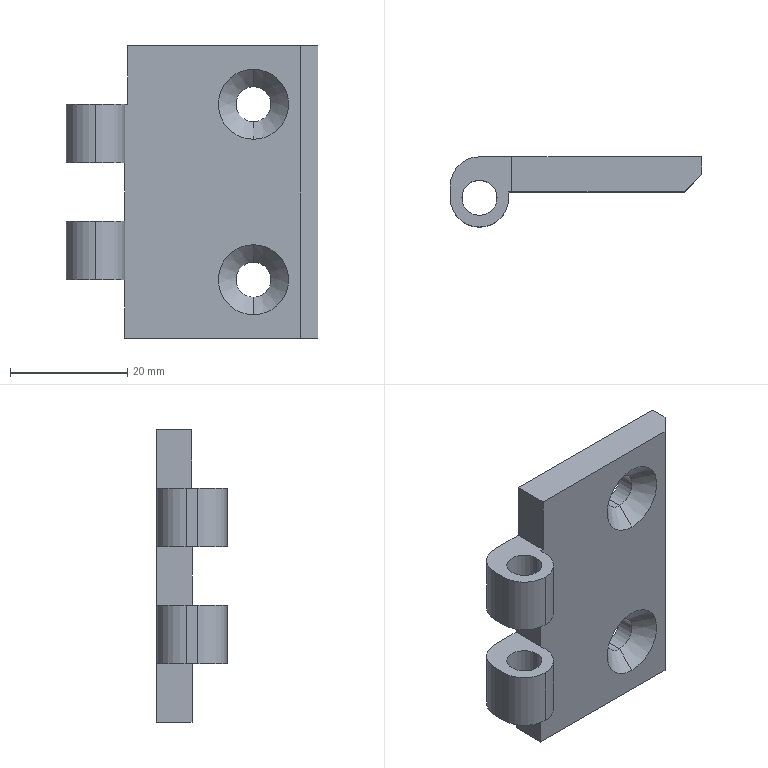Component | SolidWorks | OuterDoorHingeAssembly1-1_OuterHinge4-1 | 1 solid | 35 faces | box 43 x 12 x 50 mm | volume 10590 mm3 | plane 17 | cylinder 14 | cone 4 | commonest cylinder face diameters 6 x8 10 x6
STEP:
#1=COLOUR_RGB('',0.7922,0.8196,0.9333);
#2=FILL_AREA_STYLE_COLOUR('',#1);
#3=FILL_AREA_STYLE('',(#2));
#4=SURFACE_STYLE_FILL_AREA(#3);
#5=SURFACE_SIDE_STYLE('',(#4));
#6=SURFACE_STYLE_USAGE(.BOTH.,#5);
#7=PRESENTATION_STYLE_ASSIGNMENT((#6));
#8=CARTESIAN_POINT('',(3.383,-20.239,-59.646));
#9=VERTEX_POINT('',#8);
#10=CARTESIAN_POINT('',(3.383,-20.239,-59.409));
#11=VERTEX_POINT('',#10);
#12=CARTESIAN_POINT('',(3.383,-20.239,-59.528));
#13=DIRECTION('',(0.,-1.,0.));
#14=DIRECTION('',(-0.,0.,1.));
#15=AXIS2_PLACEMENT_3D('',#12,#13,#14);
#16=CIRCLE('',#15,0.1181);
#17=EDGE_CURVE('',#9,#11,#16,.T.);
#18=ORIENTED_EDGE('',*,*,#17,.F.);
#19=CARTESIAN_POINT('',(3.383,-20.357,-59.764));
#20=VERTEX_POINT('',#19);
#21=CARTESIAN_POINT('',(3.383,-20.239,-59.646));
#22=DIRECTION('',(0.,-0.7071,-0.7071));
#23=VECTOR('',#22,39.37);
#24=LINE('',#21,#23);
#25=EDGE_CURVE('',#9,#20,#24,.T.);
#26=ORIENTED_EDGE('',*,*,#25,.T.);
#27=CARTESIAN_POINT('',(3.383,-20.357,-59.291));
#28=VERTEX_POINT('',#27);
#29=CARTESIAN_POINT('',(3.383,-20.357,-59.528));
#30=DIRECTION('',(-0.,1.,-0.));
#31=DIRECTION('',(-0.,0.,1.));
#32=AXIS2_PLACEMENT_3D('',#29,#30,#31);
#33=CIRCLE('',#32,0.2362);
#34=EDGE_CURVE('',#28,#20,#33,.T.);
#35=ORIENTED_EDGE('',*,*,#34,.F.);
#36=CARTESIAN_POINT('',(3.383,-20.239,-59.409));
#37=DIRECTION('',(-0.,-0.7071,0.7071));
#38=VECTOR('',#37,39.37);
#39=LINE('',#36,#38);
#40=EDGE_CURVE('',#11,#28,#39,.T.);
#41=ORIENTED_EDGE('',*,*,#40,.F.);
#42=EDGE_LOOP('',(#18,#26,#35,#41));
#43=FACE_OUTER_BOUND('',#42,.T.);
#44=CARTESIAN_POINT('',(3.383,-20.239,-59.528));
#45=DIRECTION('',(0.,-1.,0.));
#46=DIRECTION('',(-0.,0.,1.));
#47=AXIS2_PLACEMENT_3D('',#44,#45,#46);
#48=CONICAL_SURFACE('',#47,0.1181,0.7854);
#49=ADVANCED_FACE('',(#43),#48,.F.);
#50=CARTESIAN_POINT('',(3.383,-20.239,-58.465));
#51=VERTEX_POINT('',#50);
#52=CARTESIAN_POINT('',(3.383,-20.239,-58.228));
#53=VERTEX_POINT('',#52);
#54=CARTESIAN_POINT('',(3.383,-20.239,-58.346));
#55=DIRECTION('',(0.,-1.,0.));
#56=DIRECTION('',(-0.,0.,1.));
#57=AXIS2_PLACEMENT_3D('',#54,#55,#56);
#58=CIRCLE('',#57,0.1181);
#59=EDGE_CURVE('',#51,#53,#58,.T.);
#60=ORIENTED_EDGE('',*,*,#59,.F.);
#61=CARTESIAN_POINT('',(3.383,-20.357,-58.583));
#62=VERTEX_POINT('',#61);
#63=CARTESIAN_POINT('',(3.383,-20.239,-58.465));
#64=DIRECTION('',(0.,-0.7071,-0.7071));
#65=VECTOR('',#64,39.37);
#66=LINE('',#63,#65);
#67=EDGE_CURVE('',#51,#62,#66,.T.);
#68=ORIENTED_EDGE('',*,*,#67,.T.);
#69=CARTESIAN_POINT('',(3.383,-20.357,-58.11));
#70=VERTEX_POINT('',#69);
#71=CARTESIAN_POINT('',(3.383,-20.357,-58.346));
#72=DIRECTION('',(-0.,1.,-0.));
#73=DIRECTION('',(-0.,0.,1.));
#74=AXIS2_PLACEMENT_3D('',#71,#72,#73);
#75=CIRCLE('',#74,0.2362);
#76=EDGE_CURVE('',#70,#62,#75,.T.);
#77=ORIENTED_EDGE('',*,*,#76,.F.);
#78=CARTESIAN_POINT('',(3.383,-20.239,-58.228));
#79=DIRECTION('',(-0.,-0.7071,0.7071));
#80=VECTOR('',#79,39.37);
#81=LINE('',#78,#80);
#82=EDGE_CURVE('',#53,#70,#81,.T.);
#83=ORIENTED_EDGE('',*,*,#82,.F.);
#84=EDGE_LOOP('',(#60,#68,#77,#83));
#85=FACE_OUTER_BOUND('',#84,.T.);
#86=CARTESIAN_POINT('',(3.383,-20.239,-58.346));
#87=DIRECTION('',(0.,-1.,0.));
#88=DIRECTION('',(-0.,0.,1.));
#89=AXIS2_PLACEMENT_3D('',#86,#87,#88);
#90=CONICAL_SURFACE('',#89,0.1181,0.7854);
#91=ADVANCED_FACE('',(#85),#90,.F.);
#92=CARTESIAN_POINT('',(3.383,-20.121,-59.646));
#93=VERTEX_POINT('',#92);
#94=CARTESIAN_POINT('',(3.383,-20.121,-59.409));
#95=VERTEX_POINT('',#94);
#96=CARTESIAN_POINT('',(3.383,-20.121,-59.528));
#97=DIRECTION('',(0.,-1.,0.));
#98=DIRECTION('',(-0.,0.,1.));
#99=AXIS2_PLACEMENT_3D('',#96,#97,#98);
#100=CIRCLE('',#99,0.1181);
#101=EDGE_CURVE('',#93,#95,#100,.T.);
#102=ORIENTED_EDGE('',*,*,#101,.F.);
#103=CARTESIAN_POINT('',(3.383,-19.964,-59.646));
#104=DIRECTION('',(0.,-1.,0.));
#105=VECTOR('',#104,39.37);
#106=LINE('',#103,#105);
#107=EDGE_CURVE('',#93,#9,#106,.T.);
#108=ORIENTED_EDGE('',*,*,#107,.T.);
#109=ORIENTED_EDGE('',*,*,#17,.T.);
#110=CARTESIAN_POINT('',(3.383,-19.964,-59.409));
#111=DIRECTION('',(0.,-1.,0.));
#112=VECTOR('',#111,39.37);
#113=LINE('',#110,#112);
#114=EDGE_CURVE('',#95,#11,#113,.T.);
#115=ORIENTED_EDGE('',*,*,#114,.F.);
#116=EDGE_LOOP('',(#102,#108,#109,#115));
#117=FACE_OUTER_BOUND('',#116,.T.);
#118=CARTESIAN_POINT('',(3.383,-19.964,-59.528));
#119=DIRECTION('',(0.,-1.,0.));
#120=DIRECTION('',(-0.,0.,1.));
#121=AXIS2_PLACEMENT_3D('',#118,#119,#120);
#122=CYLINDRICAL_SURFACE('',#121,0.1181);
#123=ADVANCED_FACE('',(#117),#122,.F.);
#124=CARTESIAN_POINT('',(3.383,-20.121,-58.465));
#125=VERTEX_POINT('',#124);
#126=CARTESIAN_POINT('',(3.383,-20.121,-58.228));
#127=VERTEX_POINT('',#126);
#128=CARTESIAN_POINT('',(3.383,-20.121,-58.346));
#129=DIRECTION('',(0.,-1.,0.));
#130=DIRECTION('',(-0.,0.,1.));
#131=AXIS2_PLACEMENT_3D('',#128,#129,#130);
#132=CIRCLE('',#131,0.1181);
#133=EDGE_CURVE('',#125,#127,#132,.T.);
#134=ORIENTED_EDGE('',*,*,#133,.F.);
#135=CARTESIAN_POINT('',(3.383,-19.964,-58.465));
#136=DIRECTION('',(0.,-1.,0.));
#137=VECTOR('',#136,39.37);
#138=LINE('',#135,#137);
#139=EDGE_CURVE('',#125,#51,#138,.T.);
#140=ORIENTED_EDGE('',*,*,#139,.T.);
#141=ORIENTED_EDGE('',*,*,#59,.T.);
#142=CARTESIAN_POINT('',(3.383,-19.964,-58.228));
#143=DIRECTION('',(0.,-1.,0.));
#144=VECTOR('',#143,39.37);
#145=LINE('',#142,#144);
#146=EDGE_CURVE('',#127,#53,#145,.T.);
#147=ORIENTED_EDGE('',*,*,#146,.F.);
#148=EDGE_LOOP('',(#134,#140,#141,#147));
#149=FACE_OUTER_BOUND('',#148,.T.);
#150=CARTESIAN_POINT('',(3.383,-19.964,-58.346));
#151=DIRECTION('',(0.,-1.,0.));
#152=DIRECTION('',(-0.,0.,1.));
#153=AXIS2_PLACEMENT_3D('',#150,#151,#152);
#154=CYLINDRICAL_SURFACE('',#153,0.1181);
#155=ADVANCED_FACE('',(#149),#154,.F.);
#156=CARTESIAN_POINT('',(2.202,-20.397,-59.528));
#157=VERTEX_POINT('',#156);
#158=CARTESIAN_POINT('',(2.438,-20.397,-59.528));
#159=VERTEX_POINT('',#158);
#160=CARTESIAN_POINT('',(2.32,-20.397,-59.528));
#161=DIRECTION('',(0.,-0.,-1.));
#162=DIRECTION('',(-1.,0.,0.));
#163=AXIS2_PLACEMENT_3D('',#160,#161,#162);
#164=CIRCLE('',#163,0.1181);
#165=EDGE_CURVE('',#157,#159,#164,.T.);
#166=ORIENTED_EDGE('',*,*,#165,.T.);
#167=CARTESIAN_POINT('',(2.438,-20.397,-59.134));
#168=VERTEX_POINT('',#167);
#169=CARTESIAN_POINT('',(2.438,-20.397,-60.315));
#170=DIRECTION('',(-0.,0.,1.));
#171=VECTOR('',#170,39.37);
#172=LINE('',#169,#171);
#173=EDGE_CURVE('',#159,#168,#172,.T.);
#174=ORIENTED_EDGE('',*,*,#173,.T.);
#175=CARTESIAN_POINT('',(2.202,-20.397,-59.134));
#176=VERTEX_POINT('',#175);
#177=CARTESIAN_POINT('',(2.32,-20.397,-59.134));
#178=DIRECTION('',(-0.,0.,1.));
#179=DIRECTION('',(1.,0.,0.));
#180=AXIS2_PLACEMENT_3D('',#177,#178,#179);
#181=CIRCLE('',#180,0.1181);
#182=EDGE_CURVE('',#168,#176,#181,.T.);
#183=ORIENTED_EDGE('',*,*,#182,.T.);
#184=CARTESIAN_POINT('',(2.202,-20.397,-60.315));
#185=DIRECTION('',(-0.,0.,1.));
#186=VECTOR('',#185,39.37);
#187=LINE('',#184,#186);
#188=EDGE_CURVE('',#157,#176,#187,.T.);
#189=ORIENTED_EDGE('',*,*,#188,.F.);
#190=EDGE_LOOP('',(#166,#174,#183,#189));
#191=FACE_OUTER_BOUND('',#190,.T.);
#192=CARTESIAN_POINT('',(2.32,-20.397,-60.315));
#193=DIRECTION('',(-0.,0.,1.));
#194=DIRECTION('',(-1.,0.,0.));
#195=AXIS2_PLACEMENT_3D('',#192,#193,#194);
#196=CYLINDRICAL_SURFACE('',#195,0.1181);
#197=ADVANCED_FACE('',(#191),#196,.F.);
#198=CARTESIAN_POINT('',(2.202,-20.397,-58.74));
#199=VERTEX_POINT('',#198);
#200=CARTESIAN_POINT('',(2.438,-20.397,-58.74));
#201=VERTEX_POINT('',#200);
#202=CARTESIAN_POINT('',(2.32,-20.397,-58.74));
#203=DIRECTION('',(0.,-0.,-1.));
#204=DIRECTION('',(-1.,0.,0.));
#205=AXIS2_PLACEMENT_3D('',#202,#203,#204);
#206=CIRCLE('',#205,0.1181);
#207=EDGE_CURVE('',#199,#201,#206,.T.);
#208=ORIENTED_EDGE('',*,*,#207,.T.);
#209=CARTESIAN_POINT('',(2.438,-20.397,-58.346));
#210=VERTEX_POINT('',#209);
#211=CARTESIAN_POINT('',(2.438,-20.397,-60.315));
#212=DIRECTION('',(-0.,0.,1.));
#213=VECTOR('',#212,39.37);
#214=LINE('',#211,#213);
#215=EDGE_CURVE('',#201,#210,#214,.T.);
#216=ORIENTED_EDGE('',*,*,#215,.T.);
#217=CARTESIAN_POINT('',(2.202,-20.397,-58.346));
#218=VERTEX_POINT('',#217);
#219=CARTESIAN_POINT('',(2.32,-20.397,-58.346));
#220=DIRECTION('',(-0.,0.,1.));
#221=DIRECTION('',(1.,0.,0.));
#222=AXIS2_PLACEMENT_3D('',#219,#220,#221);
#223=CIRCLE('',#222,0.1181);
#224=EDGE_CURVE('',#210,#218,#223,.T.);
#225=ORIENTED_EDGE('',*,*,#224,.T.);
#226=CARTESIAN_POINT('',(2.202,-20.397,-60.315));
#227=DIRECTION('',(-0.,0.,1.));
#228=VECTOR('',#227,39.37);
#229=LINE('',#226,#228);
#230=EDGE_CURVE('',#199,#218,#229,.T.);
#231=ORIENTED_EDGE('',*,*,#230,.F.);
#232=EDGE_LOOP('',(#208,#216,#225,#231));
#233=FACE_OUTER_BOUND('',#232,.T.);
#234=CARTESIAN_POINT('',(2.32,-20.397,-60.315));
#235=DIRECTION('',(-0.,0.,1.));
#236=DIRECTION('',(-1.,0.,0.));
#237=AXIS2_PLACEMENT_3D('',#234,#235,#236);
#238=CYLINDRICAL_SURFACE('',#237,0.1181);
#239=ADVANCED_FACE('',(#233),#238,.F.);
#240=CARTESIAN_POINT('',(2.123,-20.397,-58.74));
#241=VERTEX_POINT('',#240);
#242=CARTESIAN_POINT('',(2.123,-20.397,-58.346));
#243=VERTEX_POINT('',#242);
#244=CARTESIAN_POINT('',(2.123,-20.397,-59.921));
#245=DIRECTION('',(-0.,0.,1.));
#246=VECTOR('',#245,39.37);
#247=LINE('',#244,#246);
#248=EDGE_CURVE('',#241,#243,#247,.T.);
#249=ORIENTED_EDGE('',*,*,#248,.T.);
#250=CARTESIAN_POINT('',(2.123,-20.318,-58.346));
#251=VERTEX_POINT('',#250);
#252=CARTESIAN_POINT('',(2.123,-20.357,-58.346));
#253=DIRECTION('',(-0.,1.,-0.));
#254=VECTOR('',#253,39.37);
#255=LINE('',#252,#254);
#256=EDGE_CURVE('',#243,#251,#255,.T.);
#257=ORIENTED_EDGE('',*,*,#256,.T.);
#258=CARTESIAN_POINT('',(2.123,-20.318,-58.74));
#259=VERTEX_POINT('',#258);
#260=CARTESIAN_POINT('',(2.123,-20.318,-59.921));
#261=DIRECTION('',(0.,-0.,-1.));
#262=VECTOR('',#261,39.37);
#263=LINE('',#260,#262);
#264=EDGE_CURVE('',#251,#259,#263,.T.);
#265=ORIENTED_EDGE('',*,*,#264,.T.);
#266=CARTESIAN_POINT('',(2.123,-20.357,-58.74));
#267=DIRECTION('',(0.,-1.,0.));
#268=VECTOR('',#267,39.37);
#269=LINE('',#266,#268);
#270=EDGE_CURVE('',#259,#241,#269,.T.);
#271=ORIENTED_EDGE('',*,*,#270,.T.);
#272=EDGE_LOOP('',(#249,#257,#265,#271));
#273=FACE_OUTER_BOUND('',#272,.T.);
#274=CARTESIAN_POINT('',(2.123,-20.357,-59.921));
#275=DIRECTION('',(1.,0.,0.));
#276=DIRECTION('',(-0.,0.,1.));
#277=AXIS2_PLACEMENT_3D('',#274,#275,#276);
#278=PLANE('',#277);
#279=ADVANCED_FACE('',(#273),#278,.F.);
#280=CARTESIAN_POINT('',(2.517,-20.357,-58.74));
#281=VERTEX_POINT('',#280);
#282=CARTESIAN_POINT('',(2.517,-20.357,-58.346));
#283=VERTEX_POINT('',#282);
#284=CARTESIAN_POINT('',(2.517,-20.357,-59.921));
#285=DIRECTION('',(-0.,0.,1.));
#286=VECTOR('',#285,39.37);
#287=LINE('',#284,#286);
#288=EDGE_CURVE('',#281,#283,#287,.T.);
#289=ORIENTED_EDGE('',*,*,#288,.T.);
#290=CARTESIAN_POINT('',(2.517,-20.397,-58.346));
#291=VERTEX_POINT('',#290);
#292=CARTESIAN_POINT('',(2.517,-20.594,-58.346));
#293=DIRECTION('',(0.,-1.,0.));
#294=VECTOR('',#293,39.37);
#295=LINE('',#292,#294);
#296=EDGE_CURVE('',#283,#291,#295,.T.);
#297=ORIENTED_EDGE('',*,*,#296,.T.);
#298=CARTESIAN_POINT('',(2.517,-20.397,-58.74));
#299=VERTEX_POINT('',#298);
#300=CARTESIAN_POINT('',(2.517,-20.397,-59.921));
#301=DIRECTION('',(0.,-0.,-1.));
#302=VECTOR('',#301,39.37);
#303=LINE('',#300,#302);
#304=EDGE_CURVE('',#291,#299,#303,.T.);
#305=ORIENTED_EDGE('',*,*,#304,.T.);
#306=CARTESIAN_POINT('',(2.517,-20.712,-58.74));
#307=DIRECTION('',(-0.,1.,-0.));
#308=VECTOR('',#307,39.37);
#309=LINE('',#306,#308);
#310=EDGE_CURVE('',#299,#281,#309,.T.);
#311=ORIENTED_EDGE('',*,*,#310,.T.);
#312=EDGE_LOOP('',(#289,#297,#305,#311));
#313=FACE_OUTER_BOUND('',#312,.T.);
#314=CARTESIAN_POINT('',(2.517,-20.594,-59.921));
#315=DIRECTION('',(-1.,-0.,-0.));
#316=DIRECTION('',(0.,-0.,-1.));
#317=AXIS2_PLACEMENT_3D('',#314,#315,#316);
#318=PLANE('',#317);
#319=ADVANCED_FACE('',(#313),#318,.F.);
#320=ORIENTED_EDGE('',*,*,#215,.F.);
#321=CARTESIAN_POINT('',(2.32,-20.397,-58.74));
#322=DIRECTION('',(0.,-0.,-1.));
#323=DIRECTION('',(-1.,0.,0.));
#324=AXIS2_PLACEMENT_3D('',#321,#322,#323);
#325=CIRCLE('',#324,0.1181);
#326=EDGE_CURVE('',#201,#199,#325,.T.);
#327=ORIENTED_EDGE('',*,*,#326,.T.);
#328=ORIENTED_EDGE('',*,*,#230,.T.);
#329=CARTESIAN_POINT('',(2.32,-20.397,-58.346));
#330=DIRECTION('',(-0.,0.,1.));
#331=DIRECTION('',(1.,0.,0.));
#332=AXIS2_PLACEMENT_3D('',#329,#330,#331);
#333=CIRCLE('',#332,0.1181);
#334=EDGE_CURVE('',#218,#210,#333,.T.);
#335=ORIENTED_EDGE('',*,*,#334,.T.);
#336=EDGE_LOOP('',(#320,#327,#328,#335));
#337=FACE_OUTER_BOUND('',#336,.T.);
#338=CARTESIAN_POINT('',(2.32,-20.397,-60.315));
#339=DIRECTION('',(-0.,0.,1.));
#340=DIRECTION('',(-1.,0.,0.));
#341=AXIS2_PLACEMENT_3D('',#338,#339,#340);
#342=CYLINDRICAL_SURFACE('',#341,0.1181);
#343=ADVANCED_FACE('',(#337),#342,.F.);
#344=CARTESIAN_POINT('',(2.32,-20.121,-58.346));
#345=VERTEX_POINT('',#344);
#346=CARTESIAN_POINT('',(2.32,-20.318,-58.346));
#347=DIRECTION('',(-0.,0.,1.));
#348=DIRECTION('',(1.,0.,0.));
#349=AXIS2_PLACEMENT_3D('',#346,#347,#348);
#350=CIRCLE('',#349,0.1969);
#351=EDGE_CURVE('',#345,#251,#350,.T.);
#352=ORIENTED_EDGE('',*,*,#351,.F.);
#353=CARTESIAN_POINT('',(2.32,-20.121,-58.74));
#354=VERTEX_POINT('',#353);
#355=CARTESIAN_POINT('',(2.32,-20.121,-57.953));
#356=DIRECTION('',(-0.,0.,1.));
#357=VECTOR('',#356,39.37);
#358=LINE('',#355,#357);
#359=EDGE_CURVE('',#354,#345,#358,.T.);
#360=ORIENTED_EDGE('',*,*,#359,.F.);
#361=CARTESIAN_POINT('',(2.32,-20.318,-58.74));
#362=DIRECTION('',(0.,-0.,-1.));
#363=DIRECTION('',(-1.,0.,0.));
#364=AXIS2_PLACEMENT_3D('',#361,#362,#363);
#365=CIRCLE('',#364,0.1969);
#366=EDGE_CURVE('',#259,#354,#365,.T.);
#367=ORIENTED_EDGE('',*,*,#366,.F.);
#368=ORIENTED_EDGE('',*,*,#264,.F.);
#369=EDGE_LOOP('',(#352,#360,#367,#368));
#370=FACE_OUTER_BOUND('',#369,.T.);
#371=CARTESIAN_POINT('',(2.32,-20.318,-59.921));
#372=DIRECTION('',(0.,-0.,-1.));
#373=DIRECTION('',(1.,0.,0.));
#374=AXIS2_PLACEMENT_3D('',#371,#372,#373);
#375=CYLINDRICAL_SURFACE('',#374,0.1969);
#376=ADVANCED_FACE('',(#370),#375,.T.);
#377=CARTESIAN_POINT('',(2.32,-20.594,-58.346));
#378=VERTEX_POINT('',#377);
#379=CARTESIAN_POINT('',(2.32,-20.397,-58.346));
#380=DIRECTION('',(-0.,0.,1.));
#381=DIRECTION('',(1.,0.,0.));
#382=AXIS2_PLACEMENT_3D('',#379,#380,#381);
#383=CIRCLE('',#382,0.1969);
#384=EDGE_CURVE('',#243,#378,#383,.T.);
#385=ORIENTED_EDGE('',*,*,#384,.F.);
#386=ORIENTED_EDGE('',*,*,#248,.F.);
#387=CARTESIAN_POINT('',(2.32,-20.594,-58.74));
#388=VERTEX_POINT('',#387);
#389=CARTESIAN_POINT('',(2.32,-20.397,-58.74));
#390=DIRECTION('',(0.,-0.,-1.));
#391=DIRECTION('',(-1.,0.,0.));
#392=AXIS2_PLACEMENT_3D('',#389,#390,#391);
#393=CIRCLE('',#392,0.1969);
#394=EDGE_CURVE('',#388,#241,#393,.T.);
#395=ORIENTED_EDGE('',*,*,#394,.F.);
#396=CARTESIAN_POINT('',(2.32,-20.594,-57.953));
#397=DIRECTION('',(0.,-0.,-1.));
#398=VECTOR('',#397,39.37);
#399=LINE('',#396,#398);
#400=EDGE_CURVE('',#378,#388,#399,.T.);
#401=ORIENTED_EDGE('',*,*,#400,.F.);
#402=EDGE_LOOP('',(#385,#386,#395,#401));
#403=FACE_OUTER_BOUND('',#402,.T.);
#404=CARTESIAN_POINT('',(2.32,-20.397,-57.953));
#405=DIRECTION('',(0.,-0.,-1.));
#406=DIRECTION('',(1.,0.,0.));
#407=AXIS2_PLACEMENT_3D('',#404,#405,#406);
#408=CYLINDRICAL_SURFACE('',#407,0.1969);
#409=ADVANCED_FACE('',(#403),#408,.T.);
#410=CARTESIAN_POINT('',(2.32,-20.397,-58.346));
#411=DIRECTION('',(-0.,0.,1.));
#412=DIRECTION('',(1.,0.,0.));
#413=AXIS2_PLACEMENT_3D('',#410,#411,#412);
#414=CIRCLE('',#413,0.1969);
#415=EDGE_CURVE('',#378,#291,#414,.T.);
#416=ORIENTED_EDGE('',*,*,#415,.F.);
#417=ORIENTED_EDGE('',*,*,#400,.T.);
#418=CARTESIAN_POINT('',(2.32,-20.397,-58.74));
#419=DIRECTION('',(0.,-0.,-1.));
#420=DIRECTION('',(-1.,0.,0.));
#421=AXIS2_PLACEMENT_3D('',#418,#419,#420);
#422=CIRCLE('',#421,0.1969);
#423=EDGE_CURVE('',#299,#388,#422,.T.);
#424=ORIENTED_EDGE('',*,*,#423,.F.);
#425=ORIENTED_EDGE('',*,*,#304,.F.);
#426=EDGE_LOOP('',(#416,#417,#424,#425));
#427=FACE_OUTER_BOUND('',#426,.T.);
#428=CARTESIAN_POINT('',(2.32,-20.397,-57.953));
#429=DIRECTION('',(-0.,0.,1.));
#430=DIRECTION('',(-1.,0.,0.));
#431=AXIS2_PLACEMENT_3D('',#428,#429,#430);
#432=CYLINDRICAL_SURFACE('',#431,0.1969);
#433=ADVANCED_FACE('',(#427),#432,.T.);
#434=CARTESIAN_POINT('',(3.816,-20.239,-57.953));
#435=VERTEX_POINT('',#434);
#436=CARTESIAN_POINT('',(3.816,-20.121,-57.953));
#437=VERTEX_POINT('',#436);
#438=CARTESIAN_POINT('',(3.816,-20.357,-57.953));
#439=DIRECTION('',(-0.,1.,-0.));
#440=VECTOR('',#439,39.37);
#441=LINE('',#438,#440);
#442=EDGE_CURVE('',#435,#437,#441,.T.);
#443=ORIENTED_EDGE('',*,*,#442,.F.);
#444=CARTESIAN_POINT('',(3.816,-20.239,-59.921));
#445=VERTEX_POINT('',#444);
#446=CARTESIAN_POINT('',(3.816,-20.239,-59.921));
#447=DIRECTION('',(0.,-0.,-1.));
#448=VECTOR('',#447,39.37);
#449=LINE('',#446,#448);
#450=EDGE_CURVE('',#435,#445,#449,.T.);
#451=ORIENTED_EDGE('',*,*,#450,.T.);
#452=CARTESIAN_POINT('',(3.816,-20.121,-59.921));
#453=VERTEX_POINT('',#452);
#454=CARTESIAN_POINT('',(3.816,-20.357,-59.921));
#455=DIRECTION('',(-0.,1.,-0.));
#456=VECTOR('',#455,39.37);
#457=LINE('',#454,#456);
#458=EDGE_CURVE('',#445,#453,#457,.T.);
#459=ORIENTED_EDGE('',*,*,#458,.T.);
#460=CARTESIAN_POINT('',(3.816,-20.121,-59.921));
#461=DIRECTION('',(-0.,0.,1.));
#462=VECTOR('',#461,39.37);
#463=LINE('',#460,#462);
#464=EDGE_CURVE('',#453,#437,#463,.T.);
#465=ORIENTED_EDGE('',*,*,#464,.T.);
#466=EDGE_LOOP('',(#443,#451,#459,#465));
#467=FACE_OUTER_BOUND('',#466,.T.);
#468=CARTESIAN_POINT('',(3.816,-20.357,-59.921));
#469=DIRECTION('',(-1.,-0.,-0.));
#470=DIRECTION('',(0.,-0.,-1.));
#471=AXIS2_PLACEMENT_3D('',#468,#469,#470);
#472=PLANE('',#471);
#473=ADVANCED_FACE('',(#467),#472,.F.);
#474=CARTESIAN_POINT('',(3.698,-20.357,-57.953));
#475=VERTEX_POINT('',#474);
#476=CARTESIAN_POINT('',(2.538,-20.357,-57.953));
#477=VERTEX_POINT('',#476);
#478=CARTESIAN_POINT('',(3.816,-20.357,-57.953));
#479=DIRECTION('',(-1.,-0.,-0.));
#480=VECTOR('',#479,39.37);
#481=LINE('',#478,#480);
#482=EDGE_CURVE('',#475,#477,#481,.T.);
#483=ORIENTED_EDGE('',*,*,#482,.F.);
#484=CARTESIAN_POINT('',(3.698,-20.357,-57.953));
#485=DIRECTION('',(0.7071,0.7071,0.));
#486=VECTOR('',#485,39.37);
#487=LINE('',#484,#486);
#488=EDGE_CURVE('',#475,#435,#487,.T.);
#489=ORIENTED_EDGE('',*,*,#488,.T.);
#490=ORIENTED_EDGE('',*,*,#442,.T.);
#491=CARTESIAN_POINT('',(2.538,-20.121,-57.953));
#492=VERTEX_POINT('',#491);
#493=CARTESIAN_POINT('',(3.816,-20.121,-57.953));
#494=DIRECTION('',(-1.,-0.,-0.));
#495=VECTOR('',#494,39.37);
#496=LINE('',#493,#495);
#497=EDGE_CURVE('',#437,#492,#496,.T.);
#498=ORIENTED_EDGE('',*,*,#497,.T.);
#499=CARTESIAN_POINT('',(2.538,-20.357,-57.953));
#500=DIRECTION('',(0.,-1.,0.));
#501=VECTOR('',#500,39.37);
#502=LINE('',#499,#501);
#503=EDGE_CURVE('',#492,#477,#502,.T.);
#504=ORIENTED_EDGE('',*,*,#503,.T.);
#505=EDGE_LOOP('',(#483,#489,#490,#498,#504));
#506=FACE_OUTER_BOUND('',#505,.T.);
#507=CARTESIAN_POINT('',(3.816,-20.357,-57.953));
#508=DIRECTION('',(0.,-0.,-1.));
#509=DIRECTION('',(1.,0.,0.));
#510=AXIS2_PLACEMENT_3D('',#507,#508,#509);
#511=PLANE('',#510);
#512=ADVANCED_FACE('',(#506),#511,.F.);
#513=CARTESIAN_POINT('',(2.123,-20.397,-59.528));
#514=VERTEX_POINT('',#513);
#515=CARTESIAN_POINT('',(2.123,-20.397,-59.134));
#516=VERTEX_POINT('',#515);
#517=CARTESIAN_POINT('',(2.123,-20.397,-59.921));
#518=DIRECTION('',(-0.,0.,1.));
#519=VECTOR('',#518,39.37);
#520=LINE('',#517,#519);
#521=EDGE_CURVE('',#514,#516,#520,.T.);
#522=ORIENTED_EDGE('',*,*,#521,.T.);
#523=CARTESIAN_POINT('',(2.123,-20.318,-59.134));
#524=VERTEX_POINT('',#523);
#525=CARTESIAN_POINT('',(2.123,-20.357,-59.134));
#526=DIRECTION('',(-0.,1.,-0.));
#527=VECTOR('',#526,39.37);
#528=LINE('',#525,#527);
#529=EDGE_CURVE('',#516,#524,#528,.T.);
#530=ORIENTED_EDGE('',*,*,#529,.T.);
#531=CARTESIAN_POINT('',(2.123,-20.318,-59.528));
#532=VERTEX_POINT('',#531);
#533=CARTESIAN_POINT('',(2.123,-20.318,-59.921));
#534=DIRECTION('',(0.,-0.,-1.));
#535=VECTOR('',#534,39.37);
#536=LINE('',#533,#535);
#537=EDGE_CURVE('',#524,#532,#536,.T.);
#538=ORIENTED_EDGE('',*,*,#537,.T.);
#539=CARTESIAN_POINT('',(2.123,-20.357,-59.528));
#540=DIRECTION('',(0.,-1.,0.));
#541=VECTOR('',#540,39.37);
#542=LINE('',#539,#541);
#543=EDGE_CURVE('',#532,#514,#542,.T.);
#544=ORIENTED_EDGE('',*,*,#543,.T.);
#545=EDGE_LOOP('',(#522,#530,#538,#544));
#546=FACE_OUTER_BOUND('',#545,.T.);
#547=CARTESIAN_POINT('',(2.123,-20.357,-59.921));
#548=DIRECTION('',(1.,0.,0.));
#549=DIRECTION('',(-0.,0.,1.));
#550=AXIS2_PLACEMENT_3D('',#547,#548,#549);
#551=PLANE('',#550);
#552=ADVANCED_FACE('',(#546),#551,.F.);
#553=ORIENTED_EDGE('',*,*,#458,.F.);
#554=CARTESIAN_POINT('',(3.698,-20.357,-59.921));
#555=VERTEX_POINT('',#554);
#556=CARTESIAN_POINT('',(3.698,-20.357,-59.921));
#557=DIRECTION('',(-0.7071,-0.7071,-0.));
#558=VECTOR('',#557,39.37);
#559=LINE('',#556,#558);
#560=EDGE_CURVE('',#445,#555,#559,.T.);
#561=ORIENTED_EDGE('',*,*,#560,.T.);
#562=CARTESIAN_POINT('',(2.517,-20.357,-59.921));
#563=VERTEX_POINT('',#562);
#564=CARTESIAN_POINT('',(3.816,-20.357,-59.921));
#565=DIRECTION('',(1.,0.,0.));
#566=VECTOR('',#565,39.37);
#567=LINE('',#564,#566);
#568=EDGE_CURVE('',#563,#555,#567,.T.);
#569=ORIENTED_EDGE('',*,*,#568,.F.);
#570=CARTESIAN_POINT('',(2.517,-20.121,-59.921));
#571=VERTEX_POINT('',#570);
#572=CARTESIAN_POINT('',(2.517,-20.712,-59.921));
#573=DIRECTION('',(-0.,1.,-0.));
#574=VECTOR('',#573,39.37);
#575=LINE('',#572,#574);
#576=EDGE_CURVE('',#563,#571,#575,.T.);
#577=ORIENTED_EDGE('',*,*,#576,.T.);
#578=CARTESIAN_POINT('',(3.816,-20.121,-59.921));
#579=DIRECTION('',(1.,0.,0.));
#580=VECTOR('',#579,39.37);
#581=LINE('',#578,#580);
#582=EDGE_CURVE('',#571,#453,#581,.T.);
#583=ORIENTED_EDGE('',*,*,#582,.T.);
#584=EDGE_LOOP('',(#553,#561,#569,#577,#583));
#585=FACE_OUTER_BOUND('',#584,.T.);
#586=CARTESIAN_POINT('',(3.816,-20.357,-59.921));
#587=DIRECTION('',(-0.,0.,1.));
#588=DIRECTION('',(-1.,-0.,-0.));
#589=AXIS2_PLACEMENT_3D('',#586,#587,#588);
#590=PLANE('',#589);
#591=ADVANCED_FACE('',(#585),#590,.F.);
#592=ORIENTED_EDGE('',*,*,#76,.T.);
#593=CARTESIAN_POINT('',(3.383,-20.357,-58.346));
#594=DIRECTION('',(-0.,1.,-0.));
#595=DIRECTION('',(-0.,0.,1.));
#596=AXIS2_PLACEMENT_3D('',#593,#594,#595);
#597=CIRCLE('',#596,0.2362);
#598=EDGE_CURVE('',#62,#70,#597,.T.);
#599=ORIENTED_EDGE('',*,*,#598,.T.);
#600=EDGE_LOOP('',(#592,#599));
#601=FACE_BOUND('',#600,.T.);
#602=ORIENTED_EDGE('',*,*,#34,.T.);
#603=CARTESIAN_POINT('',(3.383,-20.357,-59.528));
#604=DIRECTION('',(-0.,1.,-0.));
#605=DIRECTION('',(-0.,0.,1.));
#606=AXIS2_PLACEMENT_3D('',#603,#604,#605);
#607=CIRCLE('',#606,0.2362);
#608=EDGE_CURVE('',#20,#28,#607,.T.);
#609=ORIENTED_EDGE('',*,*,#608,.T.);
#610=EDGE_LOOP('',(#602,#609));
#611=FACE_BOUND('',#610,.T.);
#612=ORIENTED_EDGE('',*,*,#568,.T.);
#613=CARTESIAN_POINT('',(3.698,-20.357,-57.953));
#614=DIRECTION('',(-0.,0.,1.));
#615=VECTOR('',#614,39.37);
#616=LINE('',#613,#615);
#617=EDGE_CURVE('',#555,#475,#616,.T.);
#618=ORIENTED_EDGE('',*,*,#617,.T.);
#619=ORIENTED_EDGE('',*,*,#482,.T.);
#620=CARTESIAN_POINT('',(2.538,-20.357,-58.346));
#621=VERTEX_POINT('',#620);
#622=CARTESIAN_POINT('',(2.538,-20.357,-57.953));
#623=DIRECTION('',(-0.,0.,1.));
#624=VECTOR('',#623,39.37);
#625=LINE('',#622,#624);
#626=EDGE_CURVE('',#621,#477,#625,.T.);
#627=ORIENTED_EDGE('',*,*,#626,.F.);
#628=CARTESIAN_POINT('',(3.816,-20.357,-58.346));
#629=DIRECTION('',(1.,0.,0.));
#630=VECTOR('',#629,39.37);
#631=LINE('',#628,#630);
#632=EDGE_CURVE('',#283,#621,#631,.T.);
#633=ORIENTED_EDGE('',*,*,#632,.F.);
#634=ORIENTED_EDGE('',*,*,#288,.F.);
#635=CARTESIAN_POINT('',(2.517,-20.357,-59.134));
#636=VERTEX_POINT('',#635);
#637=CARTESIAN_POINT('',(2.517,-20.357,-57.953));
#638=DIRECTION('',(-0.,0.,1.));
#639=VECTOR('',#638,39.37);
#640=LINE('',#637,#639);
#641=EDGE_CURVE('',#636,#281,#640,.T.);
#642=ORIENTED_EDGE('',*,*,#641,.F.);
#643=CARTESIAN_POINT('',(2.517,-20.357,-59.528));
#644=VERTEX_POINT('',#643);
#645=CARTESIAN_POINT('',(2.517,-20.357,-59.921));
#646=DIRECTION('',(-0.,0.,1.));
#647=VECTOR('',#646,39.37);
#648=LINE('',#645,#647);
#649=EDGE_CURVE('',#644,#636,#648,.T.);
#650=ORIENTED_EDGE('',*,*,#649,.F.);
#651=CARTESIAN_POINT('',(2.517,-20.357,-59.921));
#652=DIRECTION('',(-0.,0.,1.));
#653=VECTOR('',#652,39.37);
#654=LINE('',#651,#653);
#655=EDGE_CURVE('',#563,#644,#654,.T.);
#656=ORIENTED_EDGE('',*,*,#655,.F.);
#657=EDGE_LOOP('',(#612,#618,#619,#627,#633,#634,#642,#650,#656));
#658=FACE_OUTER_BOUND('',#657,.T.);
#659=CARTESIAN_POINT('',(3.816,-20.357,-57.953));
#660=DIRECTION('',(0.,-1.,0.));
#661=DIRECTION('',(-0.,0.,1.));
#662=AXIS2_PLACEMENT_3D('',#659,#660,#661);
#663=PLANE('',#662);
#664=ADVANCED_FACE('',(#601,#611,#658),#663,.T.);
#665=CARTESIAN_POINT('',(3.383,-20.121,-59.528));
#666=DIRECTION('',(0.,-1.,0.));
#667=DIRECTION('',(-0.,0.,1.));
#668=AXIS2_PLACEMENT_3D('',#665,#666,#667);
#669=CIRCLE('',#668,0.1181);
#670=EDGE_CURVE('',#95,#93,#669,.T.);
#671=ORIENTED_EDGE('',*,*,#670,.T.);
#672=ORIENTED_EDGE('',*,*,#101,.T.);
#673=EDGE_LOOP('',(#671,#672));
#674=FACE_BOUND('',#673,.T.);
#675=CARTESIAN_POINT('',(3.383,-20.121,-58.346));
#676=DIRECTION('',(0.,-1.,0.));
#677=DIRECTION('',(-0.,0.,1.));
#678=AXIS2_PLACEMENT_3D('',#675,#676,#677);
#679=CIRCLE('',#678,0.1181);
#680=EDGE_CURVE('',#127,#125,#679,.T.);
#681=ORIENTED_EDGE('',*,*,#680,.T.);
#682=ORIENTED_EDGE('',*,*,#133,.T.);
#683=EDGE_LOOP('',(#681,#682));
#684=FACE_BOUND('',#683,.T.);
#685=CARTESIAN_POINT('',(2.538,-20.121,-58.346));
#686=VERTEX_POINT('',#685);
#687=CARTESIAN_POINT('',(2.538,-20.121,-58.346));
#688=DIRECTION('',(-1.,-0.,-0.));
#689=VECTOR('',#688,39.37);
#690=LINE('',#687,#689);
#691=EDGE_CURVE('',#686,#345,#690,.T.);
#692=ORIENTED_EDGE('',*,*,#691,.F.);
#693=CARTESIAN_POINT('',(2.538,-20.121,-57.953));
#694=DIRECTION('',(-0.,0.,1.));
#695=VECTOR('',#694,39.37);
#696=LINE('',#693,#695);
#697=EDGE_CURVE('',#686,#492,#696,.T.);
#698=ORIENTED_EDGE('',*,*,#697,.T.);
#699=ORIENTED_EDGE('',*,*,#497,.F.);
#700=ORIENTED_EDGE('',*,*,#464,.F.);
#701=ORIENTED_EDGE('',*,*,#582,.F.);
#702=CARTESIAN_POINT('',(2.517,-20.121,-59.528));
#703=VERTEX_POINT('',#702);
#704=CARTESIAN_POINT('',(2.517,-20.121,-59.921));
#705=DIRECTION('',(0.,-0.,-1.));
#706=VECTOR('',#705,39.37);
#707=LINE('',#704,#706);
#708=EDGE_CURVE('',#703,#571,#707,.T.);
#709=ORIENTED_EDGE('',*,*,#708,.F.);
#710=CARTESIAN_POINT('',(2.32,-20.121,-59.528));
#711=VERTEX_POINT('',#710);
#712=CARTESIAN_POINT('',(2.517,-20.121,-59.528));
#713=DIRECTION('',(1.,0.,0.));
#714=VECTOR('',#713,39.37);
#715=LINE('',#712,#714);
#716=EDGE_CURVE('',#711,#703,#715,.T.);
#717=ORIENTED_EDGE('',*,*,#716,.F.);
#718=CARTESIAN_POINT('',(2.32,-20.121,-59.134));
#719=VERTEX_POINT('',#718);
#720=CARTESIAN_POINT('',(2.32,-20.121,-57.953));
#721=DIRECTION('',(-0.,0.,1.));
#722=VECTOR('',#721,39.37);
#723=LINE('',#720,#722);
#724=EDGE_CURVE('',#711,#719,#723,.T.);
#725=ORIENTED_EDGE('',*,*,#724,.T.);
#726=CARTESIAN_POINT('',(2.517,-20.121,-59.134));
#727=VERTEX_POINT('',#726);
#728=CARTESIAN_POINT('',(2.517,-20.121,-59.134));
#729=DIRECTION('',(-1.,-0.,-0.));
#730=VECTOR('',#729,39.37);
#731=LINE('',#728,#730);
#732=EDGE_CURVE('',#727,#719,#731,.T.);
#733=ORIENTED_EDGE('',*,*,#732,.F.);
#734=CARTESIAN_POINT('',(2.517,-20.121,-58.74));
#735=VERTEX_POINT('',#734);
#736=CARTESIAN_POINT('',(2.517,-20.121,-59.134));
#737=DIRECTION('',(0.,-0.,-1.));
#738=VECTOR('',#737,39.37);
#739=LINE('',#736,#738);
#740=EDGE_CURVE('',#735,#727,#739,.T.);
#741=ORIENTED_EDGE('',*,*,#740,.F.);
#742=CARTESIAN_POINT('',(2.517,-20.121,-58.74));
#743=DIRECTION('',(1.,0.,0.));
#744=VECTOR('',#743,39.37);
#745=LINE('',#742,#744);
#746=EDGE_CURVE('',#354,#735,#745,.T.);
#747=ORIENTED_EDGE('',*,*,#746,.F.);
#748=ORIENTED_EDGE('',*,*,#359,.T.);
#749=EDGE_LOOP('',(#692,#698,#699,#700,#701,#709,#717,#725,#733,#741,#747,#748));
#750=FACE_OUTER_BOUND('',#749,.T.);
#751=CARTESIAN_POINT('',(3.816,-20.121,-57.953));
#752=DIRECTION('',(0.,-1.,0.));
#753=DIRECTION('',(-0.,0.,1.));
#754=AXIS2_PLACEMENT_3D('',#751,#752,#753);
#755=PLANE('',#754);
#756=ADVANCED_FACE('',(#674,#684,#750),#755,.F.);
#757=ORIENTED_EDGE('',*,*,#649,.T.);
#758=CARTESIAN_POINT('',(2.517,-20.397,-59.134));
#759=VERTEX_POINT('',#758);
#760=CARTESIAN_POINT('',(2.517,-20.712,-59.134));
#761=DIRECTION('',(-0.,1.,-0.));
#762=VECTOR('',#761,39.37);
#763=LINE('',#760,#762);
#764=EDGE_CURVE('',#759,#636,#763,.T.);
#765=ORIENTED_EDGE('',*,*,#764,.F.);
#766=CARTESIAN_POINT('',(2.517,-20.397,-59.528));
#767=VERTEX_POINT('',#766);
#768=CARTESIAN_POINT('',(2.517,-20.397,-59.921));
#769=DIRECTION('',(0.,-0.,-1.));
#770=VECTOR('',#769,39.37);
#771=LINE('',#768,#770);
#772=EDGE_CURVE('',#759,#767,#771,.T.);
#773=ORIENTED_EDGE('',*,*,#772,.T.);
#774=CARTESIAN_POINT('',(2.517,-20.712,-59.528));
#775=DIRECTION('',(-0.,1.,-0.));
#776=VECTOR('',#775,39.37);
#777=LINE('',#774,#776);
#778=EDGE_CURVE('',#767,#644,#777,.T.);
#779=ORIENTED_EDGE('',*,*,#778,.T.);
#780=EDGE_LOOP('',(#757,#765,#773,#779));
#781=FACE_OUTER_BOUND('',#780,.T.);
#782=CARTESIAN_POINT('',(2.517,-20.594,-59.921));
#783=DIRECTION('',(-1.,-0.,-0.));
#784=DIRECTION('',(0.,-0.,-1.));
#785=AXIS2_PLACEMENT_3D('',#782,#783,#784);
#786=PLANE('',#785);
#787=ADVANCED_FACE('',(#781),#786,.F.);
#788=ORIENTED_EDGE('',*,*,#173,.F.);
#789=CARTESIAN_POINT('',(2.32,-20.397,-59.528));
#790=DIRECTION('',(0.,-0.,-1.));
#791=DIRECTION('',(-1.,0.,0.));
#792=AXIS2_PLACEMENT_3D('',#789,#790,#791);
#793=CIRCLE('',#792,0.1181);
#794=EDGE_CURVE('',#159,#157,#793,.T.);
#795=ORIENTED_EDGE('',*,*,#794,.T.);
#796=ORIENTED_EDGE('',*,*,#188,.T.);
#797=CARTESIAN_POINT('',(2.32,-20.397,-59.134));
#798=DIRECTION('',(-0.,0.,1.));
#799=DIRECTION('',(1.,-0.,0.));
#800=AXIS2_PLACEMENT_3D('',#797,#798,#799);
#801=CIRCLE('',#800,0.1181);
#802=EDGE_CURVE('',#176,#168,#801,.T.);
#803=ORIENTED_EDGE('',*,*,#802,.T.);
#804=EDGE_LOOP('',(#788,#795,#796,#803));
#805=FACE_OUTER_BOUND('',#804,.T.);
#806=CARTESIAN_POINT('',(2.32,-20.397,-60.315));
#807=DIRECTION('',(-0.,0.,1.));
#808=DIRECTION('',(-1.,0.,0.));
#809=AXIS2_PLACEMENT_3D('',#806,#807,#808);
#810=CYLINDRICAL_SURFACE('',#809,0.1181);
#811=ADVANCED_FACE('',(#805),#810,.F.);
#812=CARTESIAN_POINT('',(2.32,-20.318,-59.134));
#813=DIRECTION('',(-0.,0.,1.));
#814=DIRECTION('',(1.,0.,0.));
#815=AXIS2_PLACEMENT_3D('',#812,#813,#814);
#816=CIRCLE('',#815,0.1969);
#817=EDGE_CURVE('',#719,#524,#816,.T.);
#818=ORIENTED_EDGE('',*,*,#817,.F.);
#819=ORIENTED_EDGE('',*,*,#724,.F.);
#820=CARTESIAN_POINT('',(2.32,-20.318,-59.528));
#821=DIRECTION('',(0.,-0.,-1.));
#822=DIRECTION('',(-1.,0.,0.));
#823=AXIS2_PLACEMENT_3D('',#820,#821,#822);
#824=CIRCLE('',#823,0.1969);
#825=EDGE_CURVE('',#532,#711,#824,.T.);
#826=ORIENTED_EDGE('',*,*,#825,.F.);
#827=ORIENTED_EDGE('',*,*,#537,.F.);
#828=EDGE_LOOP('',(#818,#819,#826,#827));
#829=FACE_OUTER_BOUND('',#828,.T.);
#830=CARTESIAN_POINT('',(2.32,-20.318,-59.921));
#831=DIRECTION('',(0.,-0.,-1.));
#832=DIRECTION('',(1.,0.,0.));
#833=AXIS2_PLACEMENT_3D('',#830,#831,#832);
#834=CYLINDRICAL_SURFACE('',#833,0.1969);
#835=ADVANCED_FACE('',(#829),#834,.T.);
#836=CARTESIAN_POINT('',(2.32,-20.594,-59.134));
#837=VERTEX_POINT('',#836);
#838=CARTESIAN_POINT('',(2.32,-20.397,-59.134));
#839=DIRECTION('',(-0.,0.,1.));
#840=DIRECTION('',(1.,0.,0.));
#841=AXIS2_PLACEMENT_3D('',#838,#839,#840);
#842=CIRCLE('',#841,0.1969);
#843=EDGE_CURVE('',#516,#837,#842,.T.);
#844=ORIENTED_EDGE('',*,*,#843,.F.);
#845=ORIENTED_EDGE('',*,*,#521,.F.);
#846=CARTESIAN_POINT('',(2.32,-20.594,-59.528));
#847=VERTEX_POINT('',#846);
#848=CARTESIAN_POINT('',(2.32,-20.397,-59.528));
#849=DIRECTION('',(0.,-0.,-1.));
#850=DIRECTION('',(-1.,0.,0.));
#851=AXIS2_PLACEMENT_3D('',#848,#849,#850);
#852=CIRCLE('',#851,0.1969);
#853=EDGE_CURVE('',#847,#514,#852,.T.);
#854=ORIENTED_EDGE('',*,*,#853,.F.);
#855=CARTESIAN_POINT('',(2.32,-20.594,-57.953));
#856=DIRECTION('',(0.,-0.,-1.));
#857=VECTOR('',#856,39.37);
#858=LINE('',#855,#857);
#859=EDGE_CURVE('',#837,#847,#858,.T.);
#860=ORIENTED_EDGE('',*,*,#859,.F.);
#861=EDGE_LOOP('',(#844,#845,#854,#860));
#862=FACE_OUTER_BOUND('',#861,.T.);
#863=CARTESIAN_POINT('',(2.32,-20.397,-57.953));
#864=DIRECTION('',(0.,-0.,-1.));
#865=DIRECTION('',(1.,0.,0.));
#866=AXIS2_PLACEMENT_3D('',#863,#864,#865);
#867=CYLINDRICAL_SURFACE('',#866,0.1969);
#868=ADVANCED_FACE('',(#862),#867,.T.);
#869=CARTESIAN_POINT('',(2.32,-20.397,-59.134));
#870=DIRECTION('',(-0.,0.,1.));
#871=DIRECTION('',(1.,0.,0.));
#872=AXIS2_PLACEMENT_3D('',#869,#870,#871);
#873=CIRCLE('',#872,0.1969);
#874=EDGE_CURVE('',#837,#759,#873,.T.);
#875=ORIENTED_EDGE('',*,*,#874,.F.);
#876=ORIENTED_EDGE('',*,*,#859,.T.);
#877=CARTESIAN_POINT('',(2.32,-20.397,-59.528));
#878=DIRECTION('',(0.,-0.,-1.));
#879=DIRECTION('',(-1.,0.,0.));
#880=AXIS2_PLACEMENT_3D('',#877,#878,#879);
#881=CIRCLE('',#880,0.1969);
#882=EDGE_CURVE('',#767,#847,#881,.T.);
#883=ORIENTED_EDGE('',*,*,#882,.F.);
#884=ORIENTED_EDGE('',*,*,#772,.F.);
#885=EDGE_LOOP('',(#875,#876,#883,#884));
#886=FACE_OUTER_BOUND('',#885,.T.);
#887=CARTESIAN_POINT('',(2.32,-20.397,-57.953));
#888=DIRECTION('',(-0.,0.,1.));
#889=DIRECTION('',(-1.,0.,0.));
#890=AXIS2_PLACEMENT_3D('',#887,#888,#889);
#891=CYLINDRICAL_SURFACE('',#890,0.1969);
#892=ADVANCED_FACE('',(#886),#891,.T.);
#893=ORIENTED_EDGE('',*,*,#139,.F.);
#894=ORIENTED_EDGE('',*,*,#680,.F.);
#895=ORIENTED_EDGE('',*,*,#146,.T.);
#896=CARTESIAN_POINT('',(3.383,-20.239,-58.346));
#897=DIRECTION('',(0.,-1.,0.));
#898=DIRECTION('',(-0.,0.,1.));
#899=AXIS2_PLACEMENT_3D('',#896,#897,#898);
#900=CIRCLE('',#899,0.1181);
#901=EDGE_CURVE('',#53,#51,#900,.T.);
#902=ORIENTED_EDGE('',*,*,#901,.T.);
#903=EDGE_LOOP('',(#893,#894,#895,#902));
#904=FACE_OUTER_BOUND('',#903,.T.);
#905=CARTESIAN_POINT('',(3.383,-19.964,-58.346));
#906=DIRECTION('',(0.,-1.,0.));
#907=DIRECTION('',(-0.,0.,1.));
#908=AXIS2_PLACEMENT_3D('',#905,#906,#907);
#909=CYLINDRICAL_SURFACE('',#908,0.1181);
#910=ADVANCED_FACE('',(#904),#909,.F.);
#911=ORIENTED_EDGE('',*,*,#107,.F.);
#912=ORIENTED_EDGE('',*,*,#670,.F.);
#913=ORIENTED_EDGE('',*,*,#114,.T.);
#914=CARTESIAN_POINT('',(3.383,-20.239,-59.528));
#915=DIRECTION('',(0.,-1.,0.));
#916=DIRECTION('',(-0.,0.,1.));
#917=AXIS2_PLACEMENT_3D('',#914,#915,#916);
#918=CIRCLE('',#917,0.1181);
#919=EDGE_CURVE('',#11,#9,#918,.T.);
#920=ORIENTED_EDGE('',*,*,#919,.T.);
#921=EDGE_LOOP('',(#911,#912,#913,#920));
#922=FACE_OUTER_BOUND('',#921,.T.);
#923=CARTESIAN_POINT('',(3.383,-19.964,-59.528));
#924=DIRECTION('',(0.,-1.,0.));
#925=DIRECTION('',(-0.,0.,1.));
#926=AXIS2_PLACEMENT_3D('',#923,#924,#925);
#927=CYLINDRICAL_SURFACE('',#926,0.1181);
#928=ADVANCED_FACE('',(#922),#927,.F.);
#929=ORIENTED_EDGE('',*,*,#655,.T.);
#930=CARTESIAN_POINT('',(2.517,-20.712,-59.528));
#931=DIRECTION('',(-0.,1.,-0.));
#932=VECTOR('',#931,39.37);
#933=LINE('',#930,#932);
#934=EDGE_CURVE('',#644,#703,#933,.T.);
#935=ORIENTED_EDGE('',*,*,#934,.T.);
#936=ORIENTED_EDGE('',*,*,#708,.T.);
#937=ORIENTED_EDGE('',*,*,#576,.F.);
#938=EDGE_LOOP('',(#929,#935,#936,#937));
#939=FACE_OUTER_BOUND('',#938,.T.);
#940=CARTESIAN_POINT('',(2.517,-20.712,-59.921));
#941=DIRECTION('',(1.,0.,0.));
#942=DIRECTION('',(-0.,0.,1.));
#943=AXIS2_PLACEMENT_3D('',#940,#941,#942);
#944=PLANE('',#943);
#945=ADVANCED_FACE('',(#939),#944,.F.);
#946=ORIENTED_EDGE('',*,*,#825,.T.);
#947=ORIENTED_EDGE('',*,*,#716,.T.);
#948=ORIENTED_EDGE('',*,*,#934,.F.);
#949=ORIENTED_EDGE('',*,*,#778,.F.);
#950=ORIENTED_EDGE('',*,*,#882,.T.);
#951=ORIENTED_EDGE('',*,*,#853,.T.);
#952=ORIENTED_EDGE('',*,*,#543,.F.);
#953=EDGE_LOOP('',(#946,#947,#948,#949,#950,#951,#952));
#954=FACE_OUTER_BOUND('',#953,.T.);
#955=ORIENTED_EDGE('',*,*,#165,.F.);
#956=ORIENTED_EDGE('',*,*,#794,.F.);
#957=EDGE_LOOP('',(#955,#956));
#958=FACE_BOUND('',#957,.T.);
#959=CARTESIAN_POINT('',(2.517,-20.712,-59.528));
#960=DIRECTION('',(-0.,0.,1.));
#961=DIRECTION('',(-1.,-0.,-0.));
#962=AXIS2_PLACEMENT_3D('',#959,#960,#961);
#963=PLANE('',#962);
#964=ADVANCED_FACE('',(#954,#958),#963,.F.);
#965=ORIENTED_EDGE('',*,*,#641,.T.);
#966=CARTESIAN_POINT('',(2.517,-20.712,-58.74));
#967=DIRECTION('',(-0.,1.,-0.));
#968=VECTOR('',#967,39.37);
#969=LINE('',#966,#968);
#970=EDGE_CURVE('',#281,#735,#969,.T.);
#971=ORIENTED_EDGE('',*,*,#970,.T.);
#972=ORIENTED_EDGE('',*,*,#740,.T.);
#973=CARTESIAN_POINT('',(2.517,-20.712,-59.134));
#974=DIRECTION('',(-0.,1.,-0.));
#975=VECTOR('',#974,39.37);
#976=LINE('',#973,#975);
#977=EDGE_CURVE('',#636,#727,#976,.T.);
#978=ORIENTED_EDGE('',*,*,#977,.F.);
#979=EDGE_LOOP('',(#965,#971,#972,#978));
#980=FACE_OUTER_BOUND('',#979,.T.);
#981=CARTESIAN_POINT('',(2.517,-20.712,-59.134));
#982=DIRECTION('',(1.,0.,0.));
#983=DIRECTION('',(-0.,0.,1.));
#984=AXIS2_PLACEMENT_3D('',#981,#982,#983);
#985=PLANE('',#984);
#986=ADVANCED_FACE('',(#980),#985,.F.);
#987=ORIENTED_EDGE('',*,*,#366,.T.);
#988=ORIENTED_EDGE('',*,*,#746,.T.);
#989=ORIENTED_EDGE('',*,*,#970,.F.);
#990=ORIENTED_EDGE('',*,*,#310,.F.);
#991=ORIENTED_EDGE('',*,*,#423,.T.);
#992=ORIENTED_EDGE('',*,*,#394,.T.);
#993=ORIENTED_EDGE('',*,*,#270,.F.);
#994=EDGE_LOOP('',(#987,#988,#989,#990,#991,#992,#993));
#995=FACE_OUTER_BOUND('',#994,.T.);
#996=ORIENTED_EDGE('',*,*,#207,.F.);
#997=ORIENTED_EDGE('',*,*,#326,.F.);
#998=EDGE_LOOP('',(#996,#997));
#999=FACE_BOUND('',#998,.T.);
#1000=CARTESIAN_POINT('',(2.517,-20.712,-58.74));
#1001=DIRECTION('',(-0.,0.,1.));
#1002=DIRECTION('',(-1.,-0.,-0.));
#1003=AXIS2_PLACEMENT_3D('',#1000,#1001,#1002);
#1004=PLANE('',#1003);
#1005=ADVANCED_FACE('',(#995,#999),#1004,.F.);
#1006=ORIENTED_EDGE('',*,*,#817,.T.);
#1007=ORIENTED_EDGE('',*,*,#529,.F.);
#1008=ORIENTED_EDGE('',*,*,#843,.T.);
#1009=ORIENTED_EDGE('',*,*,#874,.T.);
#1010=ORIENTED_EDGE('',*,*,#764,.T.);
#1011=ORIENTED_EDGE('',*,*,#977,.T.);
#1012=ORIENTED_EDGE('',*,*,#732,.T.);
#1013=EDGE_LOOP('',(#1006,#1007,#1008,#1009,#1010,#1011,#1012));
#1014=FACE_OUTER_BOUND('',#1013,.T.);
#1015=ORIENTED_EDGE('',*,*,#802,.F.);
#1016=ORIENTED_EDGE('',*,*,#182,.F.);
#1017=EDGE_LOOP('',(#1015,#1016));
#1018=FACE_BOUND('',#1017,.T.);
#1019=CARTESIAN_POINT('',(2.517,-20.712,-59.134));
#1020=DIRECTION('',(0.,-0.,-1.));
#1021=DIRECTION('',(1.,0.,0.));
#1022=AXIS2_PLACEMENT_3D('',#1019,#1020,#1021);
#1023=PLANE('',#1022);
#1024=ADVANCED_FACE('',(#1014,#1018),#1023,.F.);
#1025=ORIENTED_EDGE('',*,*,#697,.F.);
#1026=CARTESIAN_POINT('',(2.538,-20.712,-58.346));
#1027=DIRECTION('',(-0.,1.,-0.));
#1028=VECTOR('',#1027,39.37);
#1029=LINE('',#1026,#1028);
#1030=EDGE_CURVE('',#621,#686,#1029,.T.);
#1031=ORIENTED_EDGE('',*,*,#1030,.F.);
#1032=ORIENTED_EDGE('',*,*,#626,.T.);
#1033=ORIENTED_EDGE('',*,*,#503,.F.);
#1034=EDGE_LOOP('',(#1025,#1031,#1032,#1033));
#1035=FACE_OUTER_BOUND('',#1034,.T.);
#1036=CARTESIAN_POINT('',(2.538,-20.712,-58.346));
#1037=DIRECTION('',(1.,0.,0.));
#1038=DIRECTION('',(-0.,0.,1.));
#1039=AXIS2_PLACEMENT_3D('',#1036,#1037,#1038);
#1040=PLANE('',#1039);
#1041=ADVANCED_FACE('',(#1035),#1040,.F.);
#1042=ORIENTED_EDGE('',*,*,#351,.T.);
#1043=ORIENTED_EDGE('',*,*,#256,.F.);
#1044=ORIENTED_EDGE('',*,*,#384,.T.);
#1045=ORIENTED_EDGE('',*,*,#415,.T.);
#1046=ORIENTED_EDGE('',*,*,#296,.F.);
#1047=ORIENTED_EDGE('',*,*,#632,.T.);
#1048=ORIENTED_EDGE('',*,*,#1030,.T.);
#1049=ORIENTED_EDGE('',*,*,#691,.T.);
#1050=EDGE_LOOP('',(#1042,#1043,#1044,#1045,#1046,#1047,#1048,#1049));
#1051=FACE_OUTER_BOUND('',#1050,.T.);
#1052=ORIENTED_EDGE('',*,*,#334,.F.);
#1053=ORIENTED_EDGE('',*,*,#224,.F.);
#1054=EDGE_LOOP('',(#1052,#1053));
#1055=FACE_BOUND('',#1054,.T.);
#1056=CARTESIAN_POINT('',(2.538,-20.712,-58.346));
#1057=DIRECTION('',(0.,-0.,-1.));
#1058=DIRECTION('',(1.,0.,0.));
#1059=AXIS2_PLACEMENT_3D('',#1056,#1057,#1058);
#1060=PLANE('',#1059);
#1061=ADVANCED_FACE('',(#1051,#1055),#1060,.F.);
#1062=ORIENTED_EDGE('',*,*,#67,.F.);
#1063=ORIENTED_EDGE('',*,*,#901,.F.);
#1064=ORIENTED_EDGE('',*,*,#82,.T.);
#1065=ORIENTED_EDGE('',*,*,#598,.F.);
#1066=EDGE_LOOP('',(#1062,#1063,#1064,#1065));
#1067=FACE_OUTER_BOUND('',#1066,.T.);
#1068=CARTESIAN_POINT('',(3.383,-20.239,-58.346));
#1069=DIRECTION('',(0.,-1.,0.));
#1070=DIRECTION('',(-0.,0.,1.));
#1071=AXIS2_PLACEMENT_3D('',#1068,#1069,#1070);
#1072=CONICAL_SURFACE('',#1071,0.1181,0.7854);
#1073=ADVANCED_FACE('',(#1067),#1072,.F.);
#1074=ORIENTED_EDGE('',*,*,#25,.F.);
#1075=ORIENTED_EDGE('',*,*,#919,.F.);
#1076=ORIENTED_EDGE('',*,*,#40,.T.);
#1077=ORIENTED_EDGE('',*,*,#608,.F.);
#1078=EDGE_LOOP('',(#1074,#1075,#1076,#1077));
#1079=FACE_OUTER_BOUND('',#1078,.T.);
#1080=CARTESIAN_POINT('',(3.383,-20.239,-59.528));
#1081=DIRECTION('',(0.,-1.,0.));
#1082=DIRECTION('',(-0.,0.,1.));
#1083=AXIS2_PLACEMENT_3D('',#1080,#1081,#1082);
#1084=CONICAL_SURFACE('',#1083,0.1181,0.7854);
#1085=ADVANCED_FACE('',(#1079),#1084,.F.);
#1086=ORIENTED_EDGE('',*,*,#560,.F.);
#1087=ORIENTED_EDGE('',*,*,#450,.F.);
#1088=ORIENTED_EDGE('',*,*,#488,.F.);
#1089=ORIENTED_EDGE('',*,*,#617,.F.);
#1090=EDGE_LOOP('',(#1086,#1087,#1088,#1089));
#1091=FACE_OUTER_BOUND('',#1090,.T.);
#1092=CARTESIAN_POINT('',(3.698,-20.357,-57.953));
#1093=DIRECTION('',(0.7071,-0.7071,0.));
#1094=DIRECTION('',(0.7071,0.7071,0.));
#1095=AXIS2_PLACEMENT_3D('',#1092,#1093,#1094);
#1096=PLANE('',#1095);
#1097=ADVANCED_FACE('',(#1091),#1096,.T.);
#1098=CLOSED_SHELL('',(#49,#91,#123,#155,#197,#239,#279,#319,#343,#376,#409,#433,#473,#512,#552,#591,#664,#756,#787,#811,#835,#868,#892,#910,#928,#945,#964,#986,#1005,#1024,#1041,#1061,#1073,#1085,#1097));
#1099=MANIFOLD_SOLID_BREP('',#1098);
#1100=STYLED_ITEM('',(#7),#1099);
#1101=PRESENTATION_LAYER_ASSIGNMENT('','',(#1100));
#1102=CARTESIAN_POINT('',(0.,0.,0.));
#1103=DIRECTION('',(0.,0.,1.));
#1104=DIRECTION('',(1.,0.,0.));
#1105=AXIS2_PLACEMENT_3D('',#1102,#1103,#1104);
#1106=(LENGTH_UNIT()NAMED_UNIT(*)SI_UNIT($,.METRE.));
#1107=LENGTH_MEASURE_WITH_UNIT(LENGTH_MEASURE(0.0254),#1106);
#1108=DIMENSIONAL_EXPONENTS(1.,0.,0.,0.,0.,0.,0.);
#1109=(CONVERSION_BASED_UNIT('',#1107)LENGTH_UNIT()NAMED_UNIT(#1108));
#1110=UNCERTAINTY_MEASURE_WITH_UNIT(LENGTH_MEASURE(0.00001),#1109,'','');
#1111=(NAMED_UNIT(*)PLANE_ANGLE_UNIT()SI_UNIT($,.RADIAN.));
#1112=(NAMED_UNIT(*)SI_UNIT($,.STERADIAN.)SOLID_ANGLE_UNIT());
#1113=(GEOMETRIC_REPRESENTATION_CONTEXT(3)GLOBAL_UNCERTAINTY_ASSIGNED_CONTEXT((#1110))GLOBAL_UNIT_ASSIGNED_CONTEXT((#1109,#1111,#1112))REPRESENTATION_CONTEXT('',''));
#1114=ADVANCED_BREP_SHAPE_REPRESENTATION('',(#1099,#1105),#1113);
#1115=(LENGTH_UNIT()NAMED_UNIT(*)SI_UNIT($,.METRE.));
#1116=LENGTH_MEASURE_WITH_UNIT(LENGTH_MEASURE(0.0254),#1115);
#1117=DIMENSIONAL_EXPONENTS(1.,0.,0.,0.,0.,0.,0.);
#1118=(CONVERSION_BASED_UNIT('',#1116)LENGTH_UNIT()NAMED_UNIT(#1117));
#1119=UNCERTAINTY_MEASURE_WITH_UNIT(LENGTH_MEASURE(0.00001),#1118,'','');
#1120=(NAMED_UNIT(*)PLANE_ANGLE_UNIT()SI_UNIT($,.RADIAN.));
#1121=(NAMED_UNIT(*)SI_UNIT($,.STERADIAN.)SOLID_ANGLE_UNIT());
#1122=(GEOMETRIC_REPRESENTATION_CONTEXT(3)GLOBAL_UNCERTAINTY_ASSIGNED_CONTEXT((#1119))GLOBAL_UNIT_ASSIGNED_CONTEXT((#1118,#1120,#1121))REPRESENTATION_CONTEXT('',''));
#1123=MECHANICAL_DESIGN_GEOMETRIC_PRESENTATION_REPRESENTATION('',(#1100),#1122);